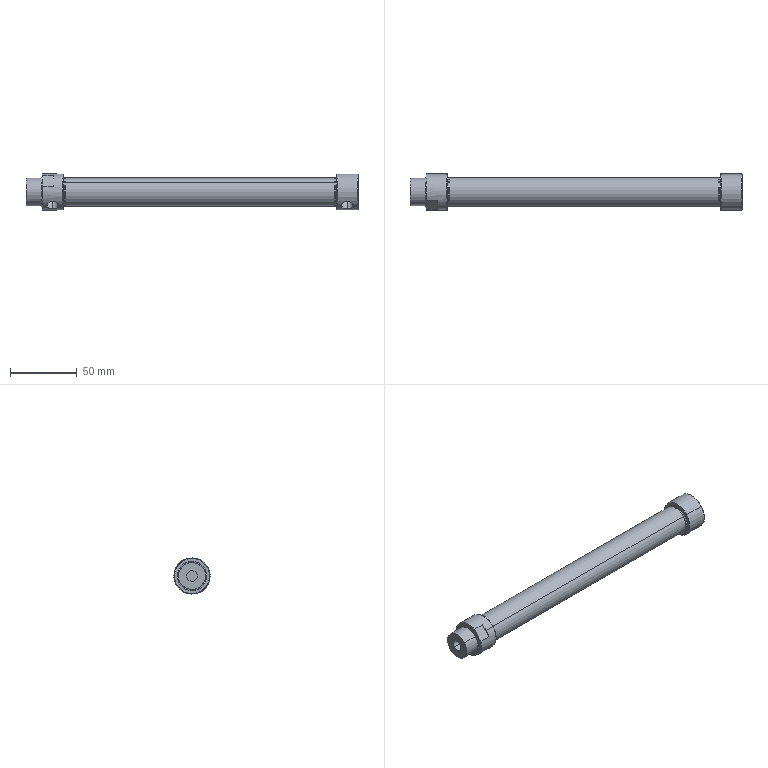Component | SolidWorks | CCDJSMA20x160SU(0)+(CS1-M-2)-1_CCDJS20MAU160 Body-1 | 1 solid | 56 faces | box 248 x 27 x 27 mm | volume 35456 mm3 | cylinder 22 | plane 16 | cone 10 | torus 8 | commonest cylinder face diameters 21.4 x6 8.566 x4 27 x4 8 x2 20 x2 20.376 x2 22 x2
build123d program:
from build123d import *

# Parameters (mm, degrees)
SKETCH2_W          = 37
SKETCH2_H          = 37
SKETCH2_W_2        = 25
SKETCH2_H_2        = 27
CUT_EXTRUDE1_DEPTH = 8.5
SKETCH1_W          = 12
SKETCH1_H          = 1.412


with BuildPart() as part:
    # Sketch1_2 → Revolve1 (revolve)
    with BuildSketch(Plane.XY, mode=Mode.PRIVATE) as revolve1_sk:
        with BuildLine():
            Line((0, 0), (0, 10.08))
            Line((0, 10.08), (0.92, 11))
            Line((0.92, 11), (12, 11))
            Line((12, 11), (12, 13.1))
            ThreePointArc((12, 13.1), (12.117, 13.383), (12.4, 13.5))
            Line((12.4, 13.5), (27.6, 13.5))
            ThreePointArc((27.6, 13.5), (27.883, 13.383), (28, 13.1))
            Line((28, 13.1), (28, 10.7))
            Line((28, 10.7), (29, 10.7))
            Line((29, 10.7), (29, 10.2))
            Line((29, 10.2), (29.3, 10.7))
            Line((29.3, 10.7), (230.7, 10.7))
            Line((230.7, 10.7), (231, 10.2))
            Line((231, 10.2), (231, 10.7))
            Line((231, 10.7), (232, 10.7))
            Line((232, 10.7), (232, 13.1))
            ThreePointArc((232, 13.1), (232.117, 13.383), (232.4, 13.5))
            Line((232.4, 13.5), (247.6, 13.5))
            ThreePointArc((247.6, 13.5), (247.883, 13.383), (248, 13.1))
            Line((248, 13.1), (248, 0))
            Line((248, 0), (0, 0))
        make_face()
    revolve(revolve1_sk.sketch.rotate(Axis((248, 0, 0), (-1, 0, 0)), 270), axis=Axis((248, 0, 0), (-1, 0, 0)))

    # Sketch2 → Cut-Extrude1 (cut)
    with BuildSketch(Plane(origin=(12, 0, 0), x_dir=(0, 0, -1), z_dir=(1, 0, 0))):
        Rectangle(SKETCH2_W, SKETCH2_H)
        Rectangle(SKETCH2_W_2, SKETCH2_H_2, mode=Mode.SUBTRACT)
    extrude(amount=CUT_EXTRUDE1_DEPTH, mode=Mode.SUBTRACT)

    # Sketch3 → Cut-Revolve1_2 (revolve, cut)
    with BuildSketch(Plane.XY, mode=Mode.PRIVATE) as cut_revolve1_2_sk:
        Polygon((20, 13.5), (24.864, 13.5), (24.283, 12.919), (24.283, 5.5), (20, 5.5), align=None)
    revolve(cut_revolve1_2_sk.sketch.rotate(Axis((20, 5.5, 0), (0, 1, 0)), 270), axis=Axis((20, 5.5, 0), (0, 1, 0)), mode=Mode.SUBTRACT)

    # Sketch4 → Cut-Revolve2 (revolve, cut)
    with BuildSketch(Plane.XY, mode=Mode.PRIVATE) as cut_revolve2_sk:
        Polygon((240, 13.5), (244.864, 13.5), (244.283, 12.919), (244.283, 5.5), (240, 5.5), align=None)
    revolve(cut_revolve2_sk.sketch.rotate(Axis((240, 5.5, 0), (0, 1, 0)), 270), axis=Axis((240, 5.5, 0), (0, 1, 0)), mode=Mode.SUBTRACT)

    # Sketch5 → Cut-Revolve3 (revolve, cut)
    with BuildSketch(Plane.XY, mode=Mode.PRIVATE) as cut_revolve3_sk:
        Polygon((0, 0), (0, 4), (39, 4), (39, 10), (221, 10), (221, 0), align=None)
    revolve(cut_revolve3_sk.sketch.rotate(Axis((221, 0, 0), (-1, 0, 0)), 270), axis=Axis((221, 0, 0), (-1, 0, 0)), mode=Mode.SUBTRACT)

    # Sketch1 → Cut-Revolve1 (revolve, cut)
    with BuildSketch(Plane.XY, mode=Mode.PRIVATE) as cut_revolve1_sk:
        with Locations((5.5, 10.894)):
            Rectangle(SKETCH1_W, SKETCH1_H)
    revolve(cut_revolve1_sk.sketch.rotate(Axis((-1.5, 0, 0), (1, 0, 0)), 90), axis=Axis((-1.5, 0, 0), (1, 0, 0)), mode=Mode.SUBTRACT)


solid = part.part

# Placed as in the assembly
solid = solid.moved(Location((96, 426.564, -63.57), (-130.678, 0, 0)))